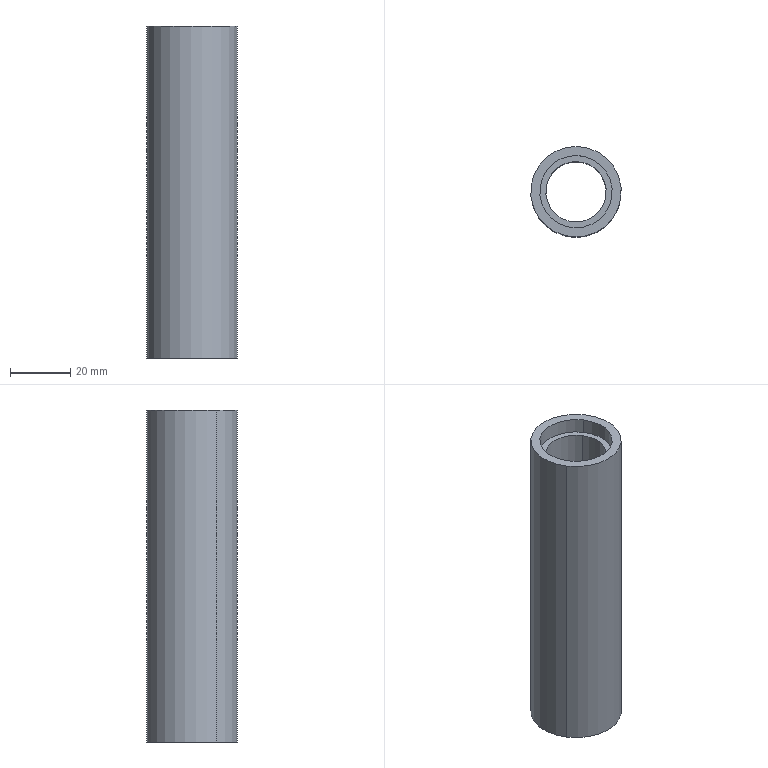Component | SolidWorks | TAR-01-39Roller-1 | 1 solid | 12 faces | box 30 x 30 x 110 mm | volume 41815 mm3 | cylinder 8 | plane 4 | commonest cylinder face diameters 24 x4 20 x2 30 x2
build123d program:
from build123d import *

# Parameters (mm, degrees)
SKETCH1_R           = 15
BOSS_EXTRUDE1_DEPTH = 110
SKETCH2_R           = 12
CUT_EXTRUDE1_DEPTH  = 5
CUT_EXTRUDE2_START  = -5
SKETCH3_R           = 12
CUT_EXTRUDE2_DEPTH  = 5
SKETCH4_R           = 10
CUT_EXTRUDE3_DEPTH  = 986


with BuildPart() as part:
    # Sketch1 → Boss-Extrude1 (new body)
    with BuildSketch(Plane.XY):
        Circle(SKETCH1_R)
    extrude(amount=BOSS_EXTRUDE1_DEPTH)

    # Sketch2 → Cut-Extrude1 (cut)
    with BuildSketch(Plane.XY.offset(110)):
        Circle(SKETCH2_R)
    extrude(amount=-CUT_EXTRUDE1_DEPTH, mode=Mode.SUBTRACT)

    # Sketch3 → Cut-Extrude2 (cut)
    with BuildSketch(Plane(origin=(0, 0, 0), x_dir=(-1, 0, 0), z_dir=(0, 0, -1)).offset(CUT_EXTRUDE2_START)):
        with Locations(Location((0, 0, 0), (0, 0, 180))):
            Circle(SKETCH3_R)
    extrude(amount=CUT_EXTRUDE2_DEPTH, mode=Mode.SUBTRACT)

    # Sketch4 → Cut-Extrude3 (cut)
    with BuildSketch(Plane(origin=(0, 0, 5), x_dir=(-1, 0, 0), z_dir=(0, 0, -1))):
        Circle(SKETCH4_R)
    extrude(amount=-CUT_EXTRUDE3_DEPTH, mode=Mode.SUBTRACT)


solid = part.part

# Placed as in the assembly
solid = solid.moved(Location((100.319, 9.938, -141.6), (0, 0, 0)))
STEP:
#1=COLOUR_RGB('',0.7922,0.8196,0.9333);
#2=FILL_AREA_STYLE_COLOUR('',#1);
#3=FILL_AREA_STYLE('',(#2));
#4=SURFACE_STYLE_FILL_AREA(#3);
#5=SURFACE_SIDE_STYLE('',(#4));
#6=SURFACE_STYLE_USAGE(.BOTH.,#5);
#7=PRESENTATION_STYLE_ASSIGNMENT((#6));
#8=CARTESIAN_POINT('',(4.279,0.6067,-5.378));
#9=VERTEX_POINT('',#8);
#10=CARTESIAN_POINT('',(3.62,0.1758,-5.378));
#11=VERTEX_POINT('',#10);
#12=CARTESIAN_POINT('',(3.95,0.3912,-5.378));
#13=DIRECTION('',(0.,0.,-1.));
#14=DIRECTION('',(-0.837,-0.5472,0.));
#15=AXIS2_PLACEMENT_3D('',#12,#13,#14);
#16=CIRCLE('',#15,0.3937);
#17=EDGE_CURVE('',#9,#11,#16,.T.);
#18=ORIENTED_EDGE('',*,*,#17,.T.);
#19=CARTESIAN_POINT('',(3.62,0.1758,-1.441));
#20=VERTEX_POINT('',#19);
#21=CARTESIAN_POINT('',(3.62,0.1758,-40.26));
#22=DIRECTION('',(0.,0.,1.));
#23=VECTOR('',#22,39.37);
#24=LINE('',#21,#23);
#25=EDGE_CURVE('',#11,#20,#24,.T.);
#26=ORIENTED_EDGE('',*,*,#25,.T.);
#27=CARTESIAN_POINT('',(4.279,0.6067,-1.441));
#28=VERTEX_POINT('',#27);
#29=CARTESIAN_POINT('',(3.95,0.3912,-1.441));
#30=DIRECTION('',(0.,0.,1.));
#31=DIRECTION('',(0.837,0.5472,0.));
#32=AXIS2_PLACEMENT_3D('',#29,#30,#31);
#33=CIRCLE('',#32,0.3937);
#34=EDGE_CURVE('',#20,#28,#33,.T.);
#35=ORIENTED_EDGE('',*,*,#34,.T.);
#36=CARTESIAN_POINT('',(4.279,0.6067,-40.26));
#37=DIRECTION('',(0.,0.,1.));
#38=VECTOR('',#37,39.37);
#39=LINE('',#36,#38);
#40=EDGE_CURVE('',#9,#28,#39,.T.);
#41=ORIENTED_EDGE('',*,*,#40,.F.);
#42=EDGE_LOOP('',(#18,#26,#35,#41));
#43=FACE_OUTER_BOUND('',#42,.T.);
#44=CARTESIAN_POINT('',(3.95,0.3912,-40.26));
#45=DIRECTION('',(0.,0.,1.));
#46=DIRECTION('',(0.837,0.5472,0.));
#47=AXIS2_PLACEMENT_3D('',#44,#45,#46);
#48=CYLINDRICAL_SURFACE('',#47,0.3937);
#49=ADVANCED_FACE('',(#43),#48,.F.);
#50=CARTESIAN_POINT('',(3.554,0.1327,-1.441));
#51=VERTEX_POINT('',#50);
#52=CARTESIAN_POINT('',(4.345,0.6498,-1.441));
#53=VERTEX_POINT('',#52);
#54=CARTESIAN_POINT('',(3.95,0.3912,-1.441));
#55=DIRECTION('',(0.,0.,1.));
#56=DIRECTION('',(0.837,0.5472,0.));
#57=AXIS2_PLACEMENT_3D('',#54,#55,#56);
#58=CIRCLE('',#57,0.4724);
#59=EDGE_CURVE('',#51,#53,#58,.T.);
#60=ORIENTED_EDGE('',*,*,#59,.F.);
#61=CARTESIAN_POINT('',(3.554,0.1327,-1.244));
#62=VERTEX_POINT('',#61);
#63=CARTESIAN_POINT('',(3.554,0.1327,-1.441));
#64=DIRECTION('',(0.,0.,1.));
#65=VECTOR('',#64,39.37);
#66=LINE('',#63,#65);
#67=EDGE_CURVE('',#51,#62,#66,.T.);
#68=ORIENTED_EDGE('',*,*,#67,.T.);
#69=CARTESIAN_POINT('',(4.345,0.6498,-1.244));
#70=VERTEX_POINT('',#69);
#71=CARTESIAN_POINT('',(3.95,0.3912,-1.244));
#72=DIRECTION('',(0.,0.,1.));
#73=DIRECTION('',(0.837,0.5472,0.));
#74=AXIS2_PLACEMENT_3D('',#71,#72,#73);
#75=CIRCLE('',#74,0.4724);
#76=EDGE_CURVE('',#62,#70,#75,.T.);
#77=ORIENTED_EDGE('',*,*,#76,.T.);
#78=CARTESIAN_POINT('',(4.345,0.6498,-1.441));
#79=DIRECTION('',(0.,0.,1.));
#80=VECTOR('',#79,39.37);
#81=LINE('',#78,#80);
#82=EDGE_CURVE('',#53,#70,#81,.T.);
#83=ORIENTED_EDGE('',*,*,#82,.F.);
#84=EDGE_LOOP('',(#60,#68,#77,#83));
#85=FACE_OUTER_BOUND('',#84,.T.);
#86=CARTESIAN_POINT('',(3.95,0.3912,-1.441));
#87=DIRECTION('',(0.,0.,1.));
#88=DIRECTION('',(0.837,0.5472,0.));
#89=AXIS2_PLACEMENT_3D('',#86,#87,#88);
#90=CYLINDRICAL_SURFACE('',#89,0.4724);
#91=ADVANCED_FACE('',(#85),#90,.F.);
#92=CARTESIAN_POINT('',(4.345,0.6498,-5.378));
#93=VERTEX_POINT('',#92);
#94=CARTESIAN_POINT('',(3.554,0.1327,-5.378));
#95=VERTEX_POINT('',#94);
#96=CARTESIAN_POINT('',(3.95,0.3912,-5.378));
#97=DIRECTION('',(0.,0.,-1.));
#98=DIRECTION('',(-0.837,-0.5472,0.));
#99=AXIS2_PLACEMENT_3D('',#96,#97,#98);
#100=CIRCLE('',#99,0.4724);
#101=EDGE_CURVE('',#93,#95,#100,.T.);
#102=ORIENTED_EDGE('',*,*,#101,.F.);
#103=CARTESIAN_POINT('',(4.345,0.6498,-5.575));
#104=VERTEX_POINT('',#103);
#105=CARTESIAN_POINT('',(4.345,0.6498,-5.378));
#106=DIRECTION('',(0.,0.,-1.));
#107=VECTOR('',#106,39.37);
#108=LINE('',#105,#107);
#109=EDGE_CURVE('',#93,#104,#108,.T.);
#110=ORIENTED_EDGE('',*,*,#109,.T.);
#111=CARTESIAN_POINT('',(3.554,0.1327,-5.575));
#112=VERTEX_POINT('',#111);
#113=CARTESIAN_POINT('',(3.95,0.3912,-5.575));
#114=DIRECTION('',(0.,0.,-1.));
#115=DIRECTION('',(-0.837,-0.5472,0.));
#116=AXIS2_PLACEMENT_3D('',#113,#114,#115);
#117=CIRCLE('',#116,0.4724);
#118=EDGE_CURVE('',#104,#112,#117,.T.);
#119=ORIENTED_EDGE('',*,*,#118,.T.);
#120=CARTESIAN_POINT('',(3.554,0.1327,-5.378));
#121=DIRECTION('',(0.,0.,-1.));
#122=VECTOR('',#121,39.37);
#123=LINE('',#120,#122);
#124=EDGE_CURVE('',#95,#112,#123,.T.);
#125=ORIENTED_EDGE('',*,*,#124,.F.);
#126=EDGE_LOOP('',(#102,#110,#119,#125));
#127=FACE_OUTER_BOUND('',#126,.T.);
#128=CARTESIAN_POINT('',(3.95,0.3912,-5.378));
#129=DIRECTION('',(0.,0.,-1.));
#130=DIRECTION('',(-0.837,-0.5472,0.));
#131=AXIS2_PLACEMENT_3D('',#128,#129,#130);
#132=CYLINDRICAL_SURFACE('',#131,0.4724);
#133=ADVANCED_FACE('',(#127),#132,.F.);
#134=CARTESIAN_POINT('',(3.455,0.06809,-5.575));
#135=VERTEX_POINT('',#134);
#136=CARTESIAN_POINT('',(4.444,0.7144,-5.575));
#137=VERTEX_POINT('',#136);
#138=CARTESIAN_POINT('',(3.95,0.3912,-5.575));
#139=DIRECTION('',(0.,0.,-1.));
#140=DIRECTION('',(-0.837,-0.5472,0.));
#141=AXIS2_PLACEMENT_3D('',#138,#139,#140);
#142=CIRCLE('',#141,0.5906);
#143=EDGE_CURVE('',#135,#137,#142,.T.);
#144=ORIENTED_EDGE('',*,*,#143,.F.);
#145=CARTESIAN_POINT('',(3.455,0.06809,-1.244));
#146=VERTEX_POINT('',#145);
#147=CARTESIAN_POINT('',(3.455,0.06809,-5.575));
#148=DIRECTION('',(0.,0.,1.));
#149=VECTOR('',#148,39.37);
#150=LINE('',#147,#149);
#151=EDGE_CURVE('',#135,#146,#150,.T.);
#152=ORIENTED_EDGE('',*,*,#151,.T.);
#153=CARTESIAN_POINT('',(4.444,0.7144,-1.244));
#154=VERTEX_POINT('',#153);
#155=CARTESIAN_POINT('',(3.95,0.3912,-1.244));
#156=DIRECTION('',(0.,0.,-1.));
#157=DIRECTION('',(-0.837,-0.5472,0.));
#158=AXIS2_PLACEMENT_3D('',#155,#156,#157);
#159=CIRCLE('',#158,0.5906);
#160=EDGE_CURVE('',#146,#154,#159,.T.);
#161=ORIENTED_EDGE('',*,*,#160,.T.);
#162=CARTESIAN_POINT('',(4.444,0.7144,-5.575));
#163=DIRECTION('',(0.,0.,1.));
#164=VECTOR('',#163,39.37);
#165=LINE('',#162,#164);
#166=EDGE_CURVE('',#137,#154,#165,.T.);
#167=ORIENTED_EDGE('',*,*,#166,.F.);
#168=EDGE_LOOP('',(#144,#152,#161,#167));
#169=FACE_OUTER_BOUND('',#168,.T.);
#170=CARTESIAN_POINT('',(3.95,0.3912,-5.575));
#171=DIRECTION('',(0.,0.,1.));
#172=DIRECTION('',(0.837,0.5472,0.));
#173=AXIS2_PLACEMENT_3D('',#170,#171,#172);
#174=CYLINDRICAL_SURFACE('',#173,0.5906);
#175=ADVANCED_FACE('',(#169),#174,.T.);
#176=ORIENTED_EDGE('',*,*,#151,.F.);
#177=CARTESIAN_POINT('',(3.95,0.3912,-5.575));
#178=DIRECTION('',(0.,0.,-1.));
#179=DIRECTION('',(-0.837,-0.5472,0.));
#180=AXIS2_PLACEMENT_3D('',#177,#178,#179);
#181=CIRCLE('',#180,0.5906);
#182=EDGE_CURVE('',#137,#135,#181,.T.);
#183=ORIENTED_EDGE('',*,*,#182,.F.);
#184=ORIENTED_EDGE('',*,*,#166,.T.);
#185=CARTESIAN_POINT('',(3.95,0.3912,-1.244));
#186=DIRECTION('',(0.,0.,-1.));
#187=DIRECTION('',(-0.837,-0.5472,0.));
#188=AXIS2_PLACEMENT_3D('',#185,#186,#187);
#189=CIRCLE('',#188,0.5906);
#190=EDGE_CURVE('',#154,#146,#189,.T.);
#191=ORIENTED_EDGE('',*,*,#190,.T.);
#192=EDGE_LOOP('',(#176,#183,#184,#191));
#193=FACE_OUTER_BOUND('',#192,.T.);
#194=CARTESIAN_POINT('',(3.95,0.3912,-5.575));
#195=DIRECTION('',(0.,0.,1.));
#196=DIRECTION('',(0.837,0.5472,0.));
#197=AXIS2_PLACEMENT_3D('',#194,#195,#196);
#198=CYLINDRICAL_SURFACE('',#197,0.5906);
#199=ADVANCED_FACE('',(#193),#198,.T.);
#200=CARTESIAN_POINT('',(3.95,0.3912,-5.575));
#201=DIRECTION('',(0.,0.,-1.));
#202=DIRECTION('',(-0.837,-0.5472,0.));
#203=AXIS2_PLACEMENT_3D('',#200,#201,#202);
#204=CIRCLE('',#203,0.4724);
#205=EDGE_CURVE('',#112,#104,#204,.T.);
#206=ORIENTED_EDGE('',*,*,#205,.F.);
#207=ORIENTED_EDGE('',*,*,#118,.F.);
#208=EDGE_LOOP('',(#206,#207));
#209=FACE_BOUND('',#208,.T.);
#210=ORIENTED_EDGE('',*,*,#182,.T.);
#211=ORIENTED_EDGE('',*,*,#143,.T.);
#212=EDGE_LOOP('',(#210,#211));
#213=FACE_OUTER_BOUND('',#212,.T.);
#214=CARTESIAN_POINT('',(3.95,0.3912,-5.575));
#215=DIRECTION('',(0.,0.,-1.));
#216=DIRECTION('',(-0.837,-0.5472,0.));
#217=AXIS2_PLACEMENT_3D('',#214,#215,#216);
#218=PLANE('',#217);
#219=ADVANCED_FACE('',(#209,#213),#218,.T.);
#220=CARTESIAN_POINT('',(3.95,0.3912,-1.244));
#221=DIRECTION('',(0.,0.,1.));
#222=DIRECTION('',(0.837,0.5472,0.));
#223=AXIS2_PLACEMENT_3D('',#220,#221,#222);
#224=CIRCLE('',#223,0.4724);
#225=EDGE_CURVE('',#70,#62,#224,.T.);
#226=ORIENTED_EDGE('',*,*,#225,.F.);
#227=ORIENTED_EDGE('',*,*,#76,.F.);
#228=EDGE_LOOP('',(#226,#227));
#229=FACE_BOUND('',#228,.T.);
#230=ORIENTED_EDGE('',*,*,#190,.F.);
#231=ORIENTED_EDGE('',*,*,#160,.F.);
#232=EDGE_LOOP('',(#230,#231));
#233=FACE_OUTER_BOUND('',#232,.T.);
#234=CARTESIAN_POINT('',(3.95,0.3912,-1.244));
#235=DIRECTION('',(0.,0.,-1.));
#236=DIRECTION('',(-0.837,-0.5472,0.));
#237=AXIS2_PLACEMENT_3D('',#234,#235,#236);
#238=PLANE('',#237);
#239=ADVANCED_FACE('',(#229,#233),#238,.F.);
#240=ORIENTED_EDGE('',*,*,#109,.F.);
#241=CARTESIAN_POINT('',(3.95,0.3912,-5.378));
#242=DIRECTION('',(0.,0.,-1.));
#243=DIRECTION('',(-0.837,-0.5472,0.));
#244=AXIS2_PLACEMENT_3D('',#241,#242,#243);
#245=CIRCLE('',#244,0.4724);
#246=EDGE_CURVE('',#95,#93,#245,.T.);
#247=ORIENTED_EDGE('',*,*,#246,.F.);
#248=ORIENTED_EDGE('',*,*,#124,.T.);
#249=ORIENTED_EDGE('',*,*,#205,.T.);
#250=EDGE_LOOP('',(#240,#247,#248,#249));
#251=FACE_OUTER_BOUND('',#250,.T.);
#252=CARTESIAN_POINT('',(3.95,0.3912,-5.378));
#253=DIRECTION('',(0.,0.,-1.));
#254=DIRECTION('',(-0.837,-0.5472,0.));
#255=AXIS2_PLACEMENT_3D('',#252,#253,#254);
#256=CYLINDRICAL_SURFACE('',#255,0.4724);
#257=ADVANCED_FACE('',(#251),#256,.F.);
#258=ORIENTED_EDGE('',*,*,#17,.F.);
#259=CARTESIAN_POINT('',(3.95,0.3912,-5.378));
#260=DIRECTION('',(0.,0.,-1.));
#261=DIRECTION('',(-0.837,-0.5472,0.));
#262=AXIS2_PLACEMENT_3D('',#259,#260,#261);
#263=CIRCLE('',#262,0.3937);
#264=EDGE_CURVE('',#11,#9,#263,.T.);
#265=ORIENTED_EDGE('',*,*,#264,.F.);
#266=EDGE_LOOP('',(#258,#265));
#267=FACE_BOUND('',#266,.T.);
#268=ORIENTED_EDGE('',*,*,#246,.T.);
#269=ORIENTED_EDGE('',*,*,#101,.T.);
#270=EDGE_LOOP('',(#268,#269));
#271=FACE_OUTER_BOUND('',#270,.T.);
#272=CARTESIAN_POINT('',(3.95,0.3912,-5.378));
#273=DIRECTION('',(0.,0.,-1.));
#274=DIRECTION('',(-0.837,-0.5472,0.));
#275=AXIS2_PLACEMENT_3D('',#272,#273,#274);
#276=PLANE('',#275);
#277=ADVANCED_FACE('',(#267,#271),#276,.T.);
#278=ORIENTED_EDGE('',*,*,#67,.F.);
#279=CARTESIAN_POINT('',(3.95,0.3912,-1.441));
#280=DIRECTION('',(0.,0.,1.));
#281=DIRECTION('',(0.837,0.5472,0.));
#282=AXIS2_PLACEMENT_3D('',#279,#280,#281);
#283=CIRCLE('',#282,0.4724);
#284=EDGE_CURVE('',#53,#51,#283,.T.);
#285=ORIENTED_EDGE('',*,*,#284,.F.);
#286=ORIENTED_EDGE('',*,*,#82,.T.);
#287=ORIENTED_EDGE('',*,*,#225,.T.);
#288=EDGE_LOOP('',(#278,#285,#286,#287));
#289=FACE_OUTER_BOUND('',#288,.T.);
#290=CARTESIAN_POINT('',(3.95,0.3912,-1.441));
#291=DIRECTION('',(0.,0.,1.));
#292=DIRECTION('',(0.837,0.5472,0.));
#293=AXIS2_PLACEMENT_3D('',#290,#291,#292);
#294=CYLINDRICAL_SURFACE('',#293,0.4724);
#295=ADVANCED_FACE('',(#289),#294,.F.);
#296=CARTESIAN_POINT('',(3.95,0.3912,-1.441));
#297=DIRECTION('',(0.,0.,1.));
#298=DIRECTION('',(0.837,0.5472,0.));
#299=AXIS2_PLACEMENT_3D('',#296,#297,#298);
#300=CIRCLE('',#299,0.3937);
#301=EDGE_CURVE('',#28,#20,#300,.T.);
#302=ORIENTED_EDGE('',*,*,#301,.F.);
#303=ORIENTED_EDGE('',*,*,#34,.F.);
#304=EDGE_LOOP('',(#302,#303));
#305=FACE_BOUND('',#304,.T.);
#306=ORIENTED_EDGE('',*,*,#284,.T.);
#307=ORIENTED_EDGE('',*,*,#59,.T.);
#308=EDGE_LOOP('',(#306,#307));
#309=FACE_OUTER_BOUND('',#308,.T.);
#310=CARTESIAN_POINT('',(3.95,0.3912,-1.441));
#311=DIRECTION('',(0.,0.,1.));
#312=DIRECTION('',(0.837,0.5472,0.));
#313=AXIS2_PLACEMENT_3D('',#310,#311,#312);
#314=PLANE('',#313);
#315=ADVANCED_FACE('',(#305,#309),#314,.T.);
#316=ORIENTED_EDGE('',*,*,#25,.F.);
#317=ORIENTED_EDGE('',*,*,#264,.T.);
#318=ORIENTED_EDGE('',*,*,#40,.T.);
#319=ORIENTED_EDGE('',*,*,#301,.T.);
#320=EDGE_LOOP('',(#316,#317,#318,#319));
#321=FACE_OUTER_BOUND('',#320,.T.);
#322=CARTESIAN_POINT('',(3.95,0.3912,-40.26));
#323=DIRECTION('',(0.,0.,1.));
#324=DIRECTION('',(0.837,0.5472,0.));
#325=AXIS2_PLACEMENT_3D('',#322,#323,#324);
#326=CYLINDRICAL_SURFACE('',#325,0.3937);
#327=ADVANCED_FACE('',(#321),#326,.F.);
#328=CLOSED_SHELL('',(#49,#91,#133,#175,#199,#219,#239,#257,#277,#295,#315,#327));
#329=MANIFOLD_SOLID_BREP('',#328);
#330=STYLED_ITEM('',(#7),#329);
#331=PRESENTATION_LAYER_ASSIGNMENT('','',(#330));
#332=CARTESIAN_POINT('',(0.,0.,0.));
#333=DIRECTION('',(0.,0.,1.));
#334=DIRECTION('',(1.,0.,0.));
#335=AXIS2_PLACEMENT_3D('',#332,#333,#334);
#336=(LENGTH_UNIT()NAMED_UNIT(*)SI_UNIT($,.METRE.));
#337=LENGTH_MEASURE_WITH_UNIT(LENGTH_MEASURE(0.0254),#336);
#338=DIMENSIONAL_EXPONENTS(1.,0.,0.,0.,0.,0.,0.);
#339=(CONVERSION_BASED_UNIT('',#337)LENGTH_UNIT()NAMED_UNIT(#338));
#340=UNCERTAINTY_MEASURE_WITH_UNIT(LENGTH_MEASURE(0.00001),#339,'','');
#341=(NAMED_UNIT(*)PLANE_ANGLE_UNIT()SI_UNIT($,.RADIAN.));
#342=(NAMED_UNIT(*)SI_UNIT($,.STERADIAN.)SOLID_ANGLE_UNIT());
#343=(GEOMETRIC_REPRESENTATION_CONTEXT(3)GLOBAL_UNCERTAINTY_ASSIGNED_CONTEXT((#340))GLOBAL_UNIT_ASSIGNED_CONTEXT((#339,#341,#342))REPRESENTATION_CONTEXT('',''));
#344=ADVANCED_BREP_SHAPE_REPRESENTATION('',(#329,#335),#343);
#345=(LENGTH_UNIT()NAMED_UNIT(*)SI_UNIT($,.METRE.));
#346=LENGTH_MEASURE_WITH_UNIT(LENGTH_MEASURE(0.0254),#345);
#347=DIMENSIONAL_EXPONENTS(1.,0.,0.,0.,0.,0.,0.);
#348=(CONVERSION_BASED_UNIT('',#346)LENGTH_UNIT()NAMED_UNIT(#347));
#349=UNCERTAINTY_MEASURE_WITH_UNIT(LENGTH_MEASURE(0.00001),#348,'','');
#350=(NAMED_UNIT(*)PLANE_ANGLE_UNIT()SI_UNIT($,.RADIAN.));
#351=(NAMED_UNIT(*)SI_UNIT($,.STERADIAN.)SOLID_ANGLE_UNIT());
#352=(GEOMETRIC_REPRESENTATION_CONTEXT(3)GLOBAL_UNCERTAINTY_ASSIGNED_CONTEXT((#349))GLOBAL_UNIT_ASSIGNED_CONTEXT((#348,#350,#351))REPRESENTATION_CONTEXT('',''));
#353=MECHANICAL_DESIGN_GEOMETRIC_PRESENTATION_REPRESENTATION('',(#330),#352);